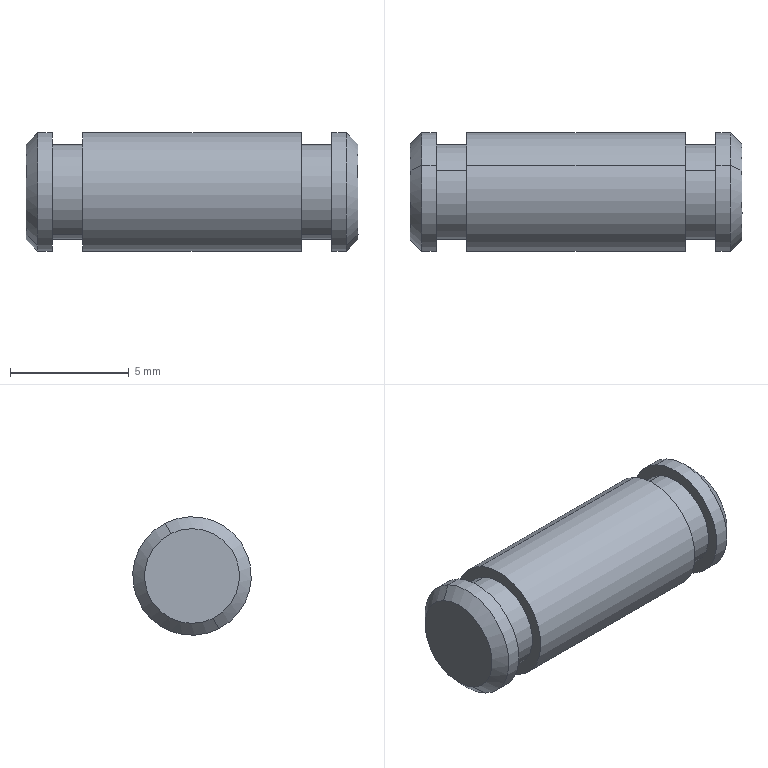Component | SolidWorks | LeverHydraulicRod22-1_HLKA-22-1 | 1 solid | 20 faces | box 14 x 5 x 5 mm | volume 253 mm3 | cylinder 10 | plane 6 | cone 4 | commonest cylinder face diameters 5 x6 4 x4
STEP:
#1=CARTESIAN_POINT('',(-2.918,4.515,-3.534));
#2=VERTEX_POINT('',#1);
#3=CARTESIAN_POINT('',(-2.918,4.426,-3.71));
#4=VERTEX_POINT('',#3);
#5=CARTESIAN_POINT('',(-2.918,4.47,-3.622));
#6=DIRECTION('',(1.,0.,0.));
#7=DIRECTION('',(0.,-0.4491,-0.8935));
#8=AXIS2_PLACEMENT_3D('',#5,#6,#7);
#9=CIRCLE('',#8,0.09843);
#10=EDGE_CURVE('',#2,#4,#9,.T.);
#11=ORIENTED_EDGE('',*,*,#10,.T.);
#12=CARTESIAN_POINT('',(-2.894,4.426,-3.71));
#13=VERTEX_POINT('',#12);
#14=CARTESIAN_POINT('',(-2.938,4.426,-3.71));
#15=DIRECTION('',(1.,0.,0.));
#16=VECTOR('',#15,39.37);
#17=LINE('',#14,#16);
#18=EDGE_CURVE('',#4,#13,#17,.T.);
#19=ORIENTED_EDGE('',*,*,#18,.T.);
#20=CARTESIAN_POINT('',(-2.894,4.515,-3.534));
#21=VERTEX_POINT('',#20);
#22=CARTESIAN_POINT('',(-2.894,4.47,-3.622));
#23=DIRECTION('',(1.,0.,0.));
#24=DIRECTION('',(0.,-0.4491,-0.8935));
#25=AXIS2_PLACEMENT_3D('',#22,#23,#24);
#26=CIRCLE('',#25,0.09843);
#27=EDGE_CURVE('',#21,#13,#26,.T.);
#28=ORIENTED_EDGE('',*,*,#27,.F.);
#29=CARTESIAN_POINT('',(-2.938,4.515,-3.534));
#30=DIRECTION('',(1.,0.,0.));
#31=VECTOR('',#30,39.37);
#32=LINE('',#29,#31);
#33=EDGE_CURVE('',#2,#21,#32,.T.);
#34=ORIENTED_EDGE('',*,*,#33,.F.);
#35=EDGE_LOOP('',(#11,#19,#28,#34));
#36=FACE_OUTER_BOUND('',#35,.T.);
#37=CARTESIAN_POINT('',(-2.938,4.47,-3.622));
#38=DIRECTION('',(1.,0.,0.));
#39=DIRECTION('',(0.,0.4491,0.8935));
#40=AXIS2_PLACEMENT_3D('',#37,#38,#39);
#41=CYLINDRICAL_SURFACE('',#40,0.09843);
#42=ADVANCED_FACE('',(#36),#41,.T.);
#43=CARTESIAN_POINT('',(-2.938,4.435,-3.692));
#44=VERTEX_POINT('',#43);
#45=CARTESIAN_POINT('',(-2.938,4.506,-3.552));
#46=VERTEX_POINT('',#45);
#47=CARTESIAN_POINT('',(-2.938,4.47,-3.622));
#48=DIRECTION('',(-1.,-0.,-0.));
#49=DIRECTION('',(0.,-0.4491,-0.8935));
#50=AXIS2_PLACEMENT_3D('',#47,#48,#49);
#51=CIRCLE('',#50,0.07874);
#52=EDGE_CURVE('',#44,#46,#51,.T.);
#53=ORIENTED_EDGE('',*,*,#52,.F.);
#54=CARTESIAN_POINT('',(-2.938,4.435,-3.692));
#55=DIRECTION('',(0.7071,-0.3176,-0.6318));
#56=VECTOR('',#55,39.37);
#57=LINE('',#54,#56);
#58=EDGE_CURVE('',#44,#4,#57,.T.);
#59=ORIENTED_EDGE('',*,*,#58,.T.);
#60=ORIENTED_EDGE('',*,*,#10,.F.);
#61=CARTESIAN_POINT('',(-2.938,4.506,-3.552));
#62=DIRECTION('',(0.7071,0.3176,0.6318));
#63=VECTOR('',#62,39.37);
#64=LINE('',#61,#63);
#65=EDGE_CURVE('',#46,#2,#64,.T.);
#66=ORIENTED_EDGE('',*,*,#65,.F.);
#67=EDGE_LOOP('',(#53,#59,#60,#66));
#68=FACE_OUTER_BOUND('',#67,.T.);
#69=CARTESIAN_POINT('',(-2.938,4.47,-3.622));
#70=DIRECTION('',(1.,0.,0.));
#71=DIRECTION('',(0.,0.4491,0.8935));
#72=AXIS2_PLACEMENT_3D('',#69,#70,#71);
#73=CONICAL_SURFACE('',#72,0.07874,0.7854);
#74=ADVANCED_FACE('',(#68),#73,.T.);
#75=CARTESIAN_POINT('',(-2.43,4.426,-3.71));
#76=VERTEX_POINT('',#75);
#77=CARTESIAN_POINT('',(-2.43,4.515,-3.534));
#78=VERTEX_POINT('',#77);
#79=CARTESIAN_POINT('',(-2.43,4.47,-3.622));
#80=DIRECTION('',(-1.,-0.,-0.));
#81=DIRECTION('',(-0.,0.4491,0.8935));
#82=AXIS2_PLACEMENT_3D('',#79,#80,#81);
#83=CIRCLE('',#82,0.09843);
#84=EDGE_CURVE('',#76,#78,#83,.T.);
#85=ORIENTED_EDGE('',*,*,#84,.F.);
#86=CARTESIAN_POINT('',(-2.406,4.426,-3.71));
#87=VERTEX_POINT('',#86);
#88=CARTESIAN_POINT('',(-2.938,4.426,-3.71));
#89=DIRECTION('',(1.,0.,0.));
#90=VECTOR('',#89,39.37);
#91=LINE('',#88,#90);
#92=EDGE_CURVE('',#76,#87,#91,.T.);
#93=ORIENTED_EDGE('',*,*,#92,.T.);
#94=CARTESIAN_POINT('',(-2.406,4.515,-3.534));
#95=VERTEX_POINT('',#94);
#96=CARTESIAN_POINT('',(-2.406,4.47,-3.622));
#97=DIRECTION('',(-1.,-0.,-0.));
#98=DIRECTION('',(0.,-0.4491,-0.8935));
#99=AXIS2_PLACEMENT_3D('',#96,#97,#98);
#100=CIRCLE('',#99,0.09843);
#101=EDGE_CURVE('',#87,#95,#100,.T.);
#102=ORIENTED_EDGE('',*,*,#101,.T.);
#103=CARTESIAN_POINT('',(-2.938,4.515,-3.534));
#104=DIRECTION('',(1.,0.,0.));
#105=VECTOR('',#104,39.37);
#106=LINE('',#103,#105);
#107=EDGE_CURVE('',#78,#95,#106,.T.);
#108=ORIENTED_EDGE('',*,*,#107,.F.);
#109=EDGE_LOOP('',(#85,#93,#102,#108));
#110=FACE_OUTER_BOUND('',#109,.T.);
#111=CARTESIAN_POINT('',(-2.938,4.47,-3.622));
#112=DIRECTION('',(1.,0.,0.));
#113=DIRECTION('',(0.,0.4491,0.8935));
#114=AXIS2_PLACEMENT_3D('',#111,#112,#113);
#115=CYLINDRICAL_SURFACE('',#114,0.09843);
#116=ADVANCED_FACE('',(#110),#115,.T.);
#117=CARTESIAN_POINT('',(-2.387,4.506,-3.552));
#118=VERTEX_POINT('',#117);
#119=CARTESIAN_POINT('',(-2.387,4.435,-3.692));
#120=VERTEX_POINT('',#119);
#121=CARTESIAN_POINT('',(-2.387,4.47,-3.622));
#122=DIRECTION('',(1.,0.,0.));
#123=DIRECTION('',(0.,-0.4491,-0.8935));
#124=AXIS2_PLACEMENT_3D('',#121,#122,#123);
#125=CIRCLE('',#124,0.07874);
#126=EDGE_CURVE('',#118,#120,#125,.T.);
#127=ORIENTED_EDGE('',*,*,#126,.F.);
#128=CARTESIAN_POINT('',(-2.406,4.515,-3.534));
#129=DIRECTION('',(-0.7071,0.3176,0.6318));
#130=VECTOR('',#129,39.37);
#131=LINE('',#128,#130);
#132=EDGE_CURVE('',#118,#95,#131,.T.);
#133=ORIENTED_EDGE('',*,*,#132,.T.);
#134=ORIENTED_EDGE('',*,*,#101,.F.);
#135=CARTESIAN_POINT('',(-2.406,4.426,-3.71));
#136=DIRECTION('',(-0.7071,-0.3176,-0.6318));
#137=VECTOR('',#136,39.37);
#138=LINE('',#135,#137);
#139=EDGE_CURVE('',#120,#87,#138,.T.);
#140=ORIENTED_EDGE('',*,*,#139,.F.);
#141=EDGE_LOOP('',(#127,#133,#134,#140));
#142=FACE_OUTER_BOUND('',#141,.T.);
#143=CARTESIAN_POINT('',(-2.406,4.47,-3.622));
#144=DIRECTION('',(-1.,-0.,-0.));
#145=DIRECTION('',(0.,-0.4491,-0.8935));
#146=AXIS2_PLACEMENT_3D('',#143,#144,#145);
#147=CONICAL_SURFACE('',#146,0.09843,0.7854);
#148=ADVANCED_FACE('',(#142),#147,.T.);
#149=CARTESIAN_POINT('',(-2.894,4.506,-3.552));
#150=VERTEX_POINT('',#149);
#151=CARTESIAN_POINT('',(-2.894,4.435,-3.692));
#152=VERTEX_POINT('',#151);
#153=CARTESIAN_POINT('',(-2.894,4.47,-3.622));
#154=DIRECTION('',(1.,0.,0.));
#155=DIRECTION('',(0.,0.4491,0.8935));
#156=AXIS2_PLACEMENT_3D('',#153,#154,#155);
#157=CIRCLE('',#156,0.07874);
#158=EDGE_CURVE('',#150,#152,#157,.T.);
#159=ORIENTED_EDGE('',*,*,#158,.T.);
#160=CARTESIAN_POINT('',(-2.843,4.435,-3.692));
#161=VERTEX_POINT('',#160);
#162=CARTESIAN_POINT('',(-2.387,4.435,-3.692));
#163=DIRECTION('',(1.,0.,0.));
#164=VECTOR('',#163,39.37);
#165=LINE('',#162,#164);
#166=EDGE_CURVE('',#152,#161,#165,.T.);
#167=ORIENTED_EDGE('',*,*,#166,.T.);
#168=CARTESIAN_POINT('',(-2.843,4.506,-3.552));
#169=VERTEX_POINT('',#168);
#170=CARTESIAN_POINT('',(-2.843,4.47,-3.622));
#171=DIRECTION('',(1.,0.,0.));
#172=DIRECTION('',(0.,0.4491,0.8935));
#173=AXIS2_PLACEMENT_3D('',#170,#171,#172);
#174=CIRCLE('',#173,0.07874);
#175=EDGE_CURVE('',#169,#161,#174,.T.);
#176=ORIENTED_EDGE('',*,*,#175,.F.);
#177=CARTESIAN_POINT('',(-2.387,4.506,-3.552));
#178=DIRECTION('',(1.,0.,0.));
#179=VECTOR('',#178,39.37);
#180=LINE('',#177,#179);
#181=EDGE_CURVE('',#150,#169,#180,.T.);
#182=ORIENTED_EDGE('',*,*,#181,.F.);
#183=EDGE_LOOP('',(#159,#167,#176,#182));
#184=FACE_OUTER_BOUND('',#183,.T.);
#185=CARTESIAN_POINT('',(-2.387,4.47,-3.622));
#186=DIRECTION('',(1.,0.,0.));
#187=DIRECTION('',(-0.,0.4491,0.8935));
#188=AXIS2_PLACEMENT_3D('',#185,#186,#187);
#189=CYLINDRICAL_SURFACE('',#188,0.07874);
#190=ADVANCED_FACE('',(#184),#189,.T.);
#191=CARTESIAN_POINT('',(-2.481,4.506,-3.552));
#192=VERTEX_POINT('',#191);
#193=CARTESIAN_POINT('',(-2.481,4.435,-3.692));
#194=VERTEX_POINT('',#193);
#195=CARTESIAN_POINT('',(-2.481,4.47,-3.622));
#196=DIRECTION('',(1.,0.,0.));
#197=DIRECTION('',(0.,0.4491,0.8935));
#198=AXIS2_PLACEMENT_3D('',#195,#196,#197);
#199=CIRCLE('',#198,0.07874);
#200=EDGE_CURVE('',#192,#194,#199,.T.);
#201=ORIENTED_EDGE('',*,*,#200,.T.);
#202=CARTESIAN_POINT('',(-2.43,4.435,-3.692));
#203=VERTEX_POINT('',#202);
#204=CARTESIAN_POINT('',(-2.387,4.435,-3.692));
#205=DIRECTION('',(1.,0.,0.));
#206=VECTOR('',#205,39.37);
#207=LINE('',#204,#206);
#208=EDGE_CURVE('',#194,#203,#207,.T.);
#209=ORIENTED_EDGE('',*,*,#208,.T.);
#210=CARTESIAN_POINT('',(-2.43,4.506,-3.552));
#211=VERTEX_POINT('',#210);
#212=CARTESIAN_POINT('',(-2.43,4.47,-3.622));
#213=DIRECTION('',(1.,0.,0.));
#214=DIRECTION('',(-0.,0.4491,0.8935));
#215=AXIS2_PLACEMENT_3D('',#212,#213,#214);
#216=CIRCLE('',#215,0.07874);
#217=EDGE_CURVE('',#211,#203,#216,.T.);
#218=ORIENTED_EDGE('',*,*,#217,.F.);
#219=CARTESIAN_POINT('',(-2.387,4.506,-3.552));
#220=DIRECTION('',(1.,0.,0.));
#221=VECTOR('',#220,39.37);
#222=LINE('',#219,#221);
#223=EDGE_CURVE('',#192,#211,#222,.T.);
#224=ORIENTED_EDGE('',*,*,#223,.F.);
#225=EDGE_LOOP('',(#201,#209,#218,#224));
#226=FACE_OUTER_BOUND('',#225,.T.);
#227=CARTESIAN_POINT('',(-2.387,4.47,-3.622));
#228=DIRECTION('',(1.,0.,0.));
#229=DIRECTION('',(-0.,0.4491,0.8935));
#230=AXIS2_PLACEMENT_3D('',#227,#228,#229);
#231=CYLINDRICAL_SURFACE('',#230,0.07874);
#232=ADVANCED_FACE('',(#226),#231,.T.);
#233=CARTESIAN_POINT('',(-2.843,4.515,-3.534));
#234=VERTEX_POINT('',#233);
#235=CARTESIAN_POINT('',(-2.843,4.426,-3.71));
#236=VERTEX_POINT('',#235);
#237=CARTESIAN_POINT('',(-2.843,4.47,-3.622));
#238=DIRECTION('',(1.,0.,0.));
#239=DIRECTION('',(0.,0.4491,0.8935));
#240=AXIS2_PLACEMENT_3D('',#237,#238,#239);
#241=CIRCLE('',#240,0.09843);
#242=EDGE_CURVE('',#234,#236,#241,.T.);
#243=ORIENTED_EDGE('',*,*,#242,.T.);
#244=CARTESIAN_POINT('',(-2.481,4.426,-3.71));
#245=VERTEX_POINT('',#244);
#246=CARTESIAN_POINT('',(-2.938,4.426,-3.71));
#247=DIRECTION('',(1.,0.,0.));
#248=VECTOR('',#247,39.37);
#249=LINE('',#246,#248);
#250=EDGE_CURVE('',#236,#245,#249,.T.);
#251=ORIENTED_EDGE('',*,*,#250,.T.);
#252=CARTESIAN_POINT('',(-2.481,4.515,-3.534));
#253=VERTEX_POINT('',#252);
#254=CARTESIAN_POINT('',(-2.481,4.47,-3.622));
#255=DIRECTION('',(-1.,-0.,-0.));
#256=DIRECTION('',(0.,-0.4491,-0.8935));
#257=AXIS2_PLACEMENT_3D('',#254,#255,#256);
#258=CIRCLE('',#257,0.09843);
#259=EDGE_CURVE('',#245,#253,#258,.T.);
#260=ORIENTED_EDGE('',*,*,#259,.T.);
#261=CARTESIAN_POINT('',(-2.938,4.515,-3.534));
#262=DIRECTION('',(1.,0.,0.));
#263=VECTOR('',#262,39.37);
#264=LINE('',#261,#263);
#265=EDGE_CURVE('',#234,#253,#264,.T.);
#266=ORIENTED_EDGE('',*,*,#265,.F.);
#267=EDGE_LOOP('',(#243,#251,#260,#266));
#268=FACE_OUTER_BOUND('',#267,.T.);
#269=CARTESIAN_POINT('',(-2.938,4.47,-3.622));
#270=DIRECTION('',(1.,0.,0.));
#271=DIRECTION('',(0.,0.4491,0.8935));
#272=AXIS2_PLACEMENT_3D('',#269,#270,#271);
#273=CYLINDRICAL_SURFACE('',#272,0.09843);
#274=ADVANCED_FACE('',(#268),#273,.T.);
#275=ORIENTED_EDGE('',*,*,#175,.T.);
#276=CARTESIAN_POINT('',(-2.843,4.47,-3.622));
#277=DIRECTION('',(1.,0.,0.));
#278=DIRECTION('',(0.,0.4491,0.8935));
#279=AXIS2_PLACEMENT_3D('',#276,#277,#278);
#280=CIRCLE('',#279,0.07874);
#281=EDGE_CURVE('',#161,#169,#280,.T.);
#282=ORIENTED_EDGE('',*,*,#281,.T.);
#283=EDGE_LOOP('',(#275,#282));
#284=FACE_BOUND('',#283,.T.);
#285=ORIENTED_EDGE('',*,*,#242,.F.);
#286=CARTESIAN_POINT('',(-2.843,4.47,-3.622));
#287=DIRECTION('',(1.,0.,0.));
#288=DIRECTION('',(0.,0.4491,0.8935));
#289=AXIS2_PLACEMENT_3D('',#286,#287,#288);
#290=CIRCLE('',#289,0.09843);
#291=EDGE_CURVE('',#236,#234,#290,.T.);
#292=ORIENTED_EDGE('',*,*,#291,.F.);
#293=EDGE_LOOP('',(#285,#292));
#294=FACE_OUTER_BOUND('',#293,.T.);
#295=CARTESIAN_POINT('',(-2.843,4.543,-3.478));
#296=DIRECTION('',(1.,-0.,0.));
#297=DIRECTION('',(0.,0.8935,-0.4491));
#298=AXIS2_PLACEMENT_3D('',#295,#296,#297);
#299=PLANE('',#298);
#300=ADVANCED_FACE('',(#284,#294),#299,.F.);
#301=ORIENTED_EDGE('',*,*,#200,.F.);
#302=CARTESIAN_POINT('',(-2.481,4.47,-3.622));
#303=DIRECTION('',(1.,0.,0.));
#304=DIRECTION('',(0.,0.4491,0.8935));
#305=AXIS2_PLACEMENT_3D('',#302,#303,#304);
#306=CIRCLE('',#305,0.07874);
#307=EDGE_CURVE('',#194,#192,#306,.T.);
#308=ORIENTED_EDGE('',*,*,#307,.F.);
#309=EDGE_LOOP('',(#301,#308));
#310=FACE_BOUND('',#309,.T.);
#311=CARTESIAN_POINT('',(-2.481,4.47,-3.622));
#312=DIRECTION('',(-1.,-0.,-0.));
#313=DIRECTION('',(0.,-0.4491,-0.8935));
#314=AXIS2_PLACEMENT_3D('',#311,#312,#313);
#315=CIRCLE('',#314,0.09843);
#316=EDGE_CURVE('',#253,#245,#315,.T.);
#317=ORIENTED_EDGE('',*,*,#316,.F.);
#318=ORIENTED_EDGE('',*,*,#259,.F.);
#319=EDGE_LOOP('',(#317,#318));
#320=FACE_OUTER_BOUND('',#319,.T.);
#321=CARTESIAN_POINT('',(-2.481,4.538,-3.487));
#322=DIRECTION('',(-1.,-0.,-0.));
#323=DIRECTION('',(0.,-0.4491,-0.8935));
#324=AXIS2_PLACEMENT_3D('',#321,#322,#323);
#325=PLANE('',#324);
#326=ADVANCED_FACE('',(#310,#320),#325,.F.);
#327=ORIENTED_EDGE('',*,*,#250,.F.);
#328=ORIENTED_EDGE('',*,*,#291,.T.);
#329=ORIENTED_EDGE('',*,*,#265,.T.);
#330=ORIENTED_EDGE('',*,*,#316,.T.);
#331=EDGE_LOOP('',(#327,#328,#329,#330));
#332=FACE_OUTER_BOUND('',#331,.T.);
#333=CARTESIAN_POINT('',(-2.938,4.47,-3.622));
#334=DIRECTION('',(1.,0.,0.));
#335=DIRECTION('',(0.,0.4491,0.8935));
#336=AXIS2_PLACEMENT_3D('',#333,#334,#335);
#337=CYLINDRICAL_SURFACE('',#336,0.09843);
#338=ADVANCED_FACE('',(#332),#337,.T.);
#339=ORIENTED_EDGE('',*,*,#208,.F.);
#340=ORIENTED_EDGE('',*,*,#307,.T.);
#341=ORIENTED_EDGE('',*,*,#223,.T.);
#342=CARTESIAN_POINT('',(-2.43,4.47,-3.622));
#343=DIRECTION('',(1.,0.,0.));
#344=DIRECTION('',(-0.,0.4491,0.8935));
#345=AXIS2_PLACEMENT_3D('',#342,#343,#344);
#346=CIRCLE('',#345,0.07874);
#347=EDGE_CURVE('',#203,#211,#346,.T.);
#348=ORIENTED_EDGE('',*,*,#347,.F.);
#349=EDGE_LOOP('',(#339,#340,#341,#348));
#350=FACE_OUTER_BOUND('',#349,.T.);
#351=CARTESIAN_POINT('',(-2.387,4.47,-3.622));
#352=DIRECTION('',(1.,0.,0.));
#353=DIRECTION('',(-0.,0.4491,0.8935));
#354=AXIS2_PLACEMENT_3D('',#351,#352,#353);
#355=CYLINDRICAL_SURFACE('',#354,0.07874);
#356=ADVANCED_FACE('',(#350),#355,.T.);
#357=ORIENTED_EDGE('',*,*,#166,.F.);
#358=CARTESIAN_POINT('',(-2.894,4.47,-3.622));
#359=DIRECTION('',(1.,0.,0.));
#360=DIRECTION('',(0.,0.4491,0.8935));
#361=AXIS2_PLACEMENT_3D('',#358,#359,#360);
#362=CIRCLE('',#361,0.07874);
#363=EDGE_CURVE('',#152,#150,#362,.T.);
#364=ORIENTED_EDGE('',*,*,#363,.T.);
#365=ORIENTED_EDGE('',*,*,#181,.T.);
#366=ORIENTED_EDGE('',*,*,#281,.F.);
#367=EDGE_LOOP('',(#357,#364,#365,#366));
#368=FACE_OUTER_BOUND('',#367,.T.);
#369=CARTESIAN_POINT('',(-2.387,4.47,-3.622));
#370=DIRECTION('',(1.,0.,0.));
#371=DIRECTION('',(-0.,0.4491,0.8935));
#372=AXIS2_PLACEMENT_3D('',#369,#370,#371);
#373=CYLINDRICAL_SURFACE('',#372,0.07874);
#374=ADVANCED_FACE('',(#368),#373,.T.);
#375=CARTESIAN_POINT('',(-2.43,4.47,-3.622));
#376=DIRECTION('',(-1.,-0.,-0.));
#377=DIRECTION('',(-0.,0.4491,0.8935));
#378=AXIS2_PLACEMENT_3D('',#375,#376,#377);
#379=CIRCLE('',#378,0.09843);
#380=EDGE_CURVE('',#78,#76,#379,.T.);
#381=ORIENTED_EDGE('',*,*,#380,.T.);
#382=ORIENTED_EDGE('',*,*,#84,.T.);
#383=EDGE_LOOP('',(#381,#382));
#384=FACE_OUTER_BOUND('',#383,.T.);
#385=ORIENTED_EDGE('',*,*,#217,.T.);
#386=ORIENTED_EDGE('',*,*,#347,.T.);
#387=EDGE_LOOP('',(#385,#386));
#388=FACE_BOUND('',#387,.T.);
#389=CARTESIAN_POINT('',(-2.43,4.365,-3.569));
#390=DIRECTION('',(1.,0.,0.));
#391=DIRECTION('',(-0.,0.4491,0.8935));
#392=AXIS2_PLACEMENT_3D('',#389,#390,#391);
#393=PLANE('',#392);
#394=ADVANCED_FACE('',(#384,#388),#393,.F.);
#395=CARTESIAN_POINT('',(-2.387,4.47,-3.622));
#396=DIRECTION('',(1.,0.,0.));
#397=DIRECTION('',(0.,-0.4491,-0.8935));
#398=AXIS2_PLACEMENT_3D('',#395,#396,#397);
#399=CIRCLE('',#398,0.07874);
#400=EDGE_CURVE('',#120,#118,#399,.T.);
#401=ORIENTED_EDGE('',*,*,#400,.T.);
#402=ORIENTED_EDGE('',*,*,#126,.T.);
#403=EDGE_LOOP('',(#401,#402));
#404=FACE_OUTER_BOUND('',#403,.T.);
#405=CARTESIAN_POINT('',(-2.387,4.47,-3.622));
#406=DIRECTION('',(-1.,-0.,-0.));
#407=DIRECTION('',(0.,-0.4491,-0.8935));
#408=AXIS2_PLACEMENT_3D('',#405,#406,#407);
#409=PLANE('',#408);
#410=ADVANCED_FACE('',(#404),#409,.F.);
#411=ORIENTED_EDGE('',*,*,#132,.F.);
#412=ORIENTED_EDGE('',*,*,#400,.F.);
#413=ORIENTED_EDGE('',*,*,#139,.T.);
#414=CARTESIAN_POINT('',(-2.406,4.47,-3.622));
#415=DIRECTION('',(-1.,-0.,-0.));
#416=DIRECTION('',(0.,-0.4491,-0.8935));
#417=AXIS2_PLACEMENT_3D('',#414,#415,#416);
#418=CIRCLE('',#417,0.09843);
#419=EDGE_CURVE('',#95,#87,#418,.T.);
#420=ORIENTED_EDGE('',*,*,#419,.F.);
#421=EDGE_LOOP('',(#411,#412,#413,#420));
#422=FACE_OUTER_BOUND('',#421,.T.);
#423=CARTESIAN_POINT('',(-2.406,4.47,-3.622));
#424=DIRECTION('',(-1.,-0.,-0.));
#425=DIRECTION('',(0.,-0.4491,-0.8935));
#426=AXIS2_PLACEMENT_3D('',#423,#424,#425);
#427=CONICAL_SURFACE('',#426,0.09843,0.7854);
#428=ADVANCED_FACE('',(#422),#427,.T.);
#429=ORIENTED_EDGE('',*,*,#92,.F.);
#430=ORIENTED_EDGE('',*,*,#380,.F.);
#431=ORIENTED_EDGE('',*,*,#107,.T.);
#432=ORIENTED_EDGE('',*,*,#419,.T.);
#433=EDGE_LOOP('',(#429,#430,#431,#432));
#434=FACE_OUTER_BOUND('',#433,.T.);
#435=CARTESIAN_POINT('',(-2.938,4.47,-3.622));
#436=DIRECTION('',(1.,0.,0.));
#437=DIRECTION('',(0.,0.4491,0.8935));
#438=AXIS2_PLACEMENT_3D('',#435,#436,#437);
#439=CYLINDRICAL_SURFACE('',#438,0.09843);
#440=ADVANCED_FACE('',(#434),#439,.T.);
#441=ORIENTED_EDGE('',*,*,#27,.T.);
#442=CARTESIAN_POINT('',(-2.894,4.47,-3.622));
#443=DIRECTION('',(1.,0.,0.));
#444=DIRECTION('',(0.,-0.4491,-0.8935));
#445=AXIS2_PLACEMENT_3D('',#442,#443,#444);
#446=CIRCLE('',#445,0.09843);
#447=EDGE_CURVE('',#13,#21,#446,.T.);
#448=ORIENTED_EDGE('',*,*,#447,.T.);
#449=EDGE_LOOP('',(#441,#448));
#450=FACE_OUTER_BOUND('',#449,.T.);
#451=ORIENTED_EDGE('',*,*,#158,.F.);
#452=ORIENTED_EDGE('',*,*,#363,.F.);
#453=EDGE_LOOP('',(#451,#452));
#454=FACE_BOUND('',#453,.T.);
#455=CARTESIAN_POINT('',(-2.894,4.4,-3.587));
#456=DIRECTION('',(-1.,-0.,-0.));
#457=DIRECTION('',(0.,-0.4491,-0.8935));
#458=AXIS2_PLACEMENT_3D('',#455,#456,#457);
#459=PLANE('',#458);
#460=ADVANCED_FACE('',(#450,#454),#459,.F.);
#461=CARTESIAN_POINT('',(-2.938,4.47,-3.622));
#462=DIRECTION('',(-1.,-0.,-0.));
#463=DIRECTION('',(0.,-0.4491,-0.8935));
#464=AXIS2_PLACEMENT_3D('',#461,#462,#463);
#465=CIRCLE('',#464,0.07874);
#466=EDGE_CURVE('',#46,#44,#465,.T.);
#467=ORIENTED_EDGE('',*,*,#466,.T.);
#468=ORIENTED_EDGE('',*,*,#52,.T.);
#469=EDGE_LOOP('',(#467,#468));
#470=FACE_OUTER_BOUND('',#469,.T.);
#471=CARTESIAN_POINT('',(-2.938,4.47,-3.622));
#472=DIRECTION('',(-1.,-0.,-0.));
#473=DIRECTION('',(0.,-0.4491,-0.8935));
#474=AXIS2_PLACEMENT_3D('',#471,#472,#473);
#475=PLANE('',#474);
#476=ADVANCED_FACE('',(#470),#475,.T.);
#477=ORIENTED_EDGE('',*,*,#58,.F.);
#478=ORIENTED_EDGE('',*,*,#466,.F.);
#479=ORIENTED_EDGE('',*,*,#65,.T.);
#480=CARTESIAN_POINT('',(-2.918,4.47,-3.622));
#481=DIRECTION('',(1.,0.,0.));
#482=DIRECTION('',(0.,-0.4491,-0.8935));
#483=AXIS2_PLACEMENT_3D('',#480,#481,#482);
#484=CIRCLE('',#483,0.09843);
#485=EDGE_CURVE('',#4,#2,#484,.T.);
#486=ORIENTED_EDGE('',*,*,#485,.F.);
#487=EDGE_LOOP('',(#477,#478,#479,#486));
#488=FACE_OUTER_BOUND('',#487,.T.);
#489=CARTESIAN_POINT('',(-2.938,4.47,-3.622));
#490=DIRECTION('',(1.,0.,0.));
#491=DIRECTION('',(0.,0.4491,0.8935));
#492=AXIS2_PLACEMENT_3D('',#489,#490,#491);
#493=CONICAL_SURFACE('',#492,0.07874,0.7854);
#494=ADVANCED_FACE('',(#488),#493,.T.);
#495=ORIENTED_EDGE('',*,*,#18,.F.);
#496=ORIENTED_EDGE('',*,*,#485,.T.);
#497=ORIENTED_EDGE('',*,*,#33,.T.);
#498=ORIENTED_EDGE('',*,*,#447,.F.);
#499=EDGE_LOOP('',(#495,#496,#497,#498));
#500=FACE_OUTER_BOUND('',#499,.T.);
#501=CARTESIAN_POINT('',(-2.938,4.47,-3.622));
#502=DIRECTION('',(1.,0.,0.));
#503=DIRECTION('',(0.,0.4491,0.8935));
#504=AXIS2_PLACEMENT_3D('',#501,#502,#503);
#505=CYLINDRICAL_SURFACE('',#504,0.09843);
#506=ADVANCED_FACE('',(#500),#505,.T.);
#507=CLOSED_SHELL('',(#42,#74,#116,#148,#190,#232,#274,#300,#326,#338,#356,#374,#394,#410,#428,#440,#460,#476,#494,#506));
#508=MANIFOLD_SOLID_BREP('',#507);
#509=CARTESIAN_POINT('',(0.,0.,0.));
#510=DIRECTION('',(0.,0.,1.));
#511=DIRECTION('',(1.,0.,0.));
#512=AXIS2_PLACEMENT_3D('',#509,#510,#511);
#513=(LENGTH_UNIT()NAMED_UNIT(*)SI_UNIT($,.METRE.));
#514=LENGTH_MEASURE_WITH_UNIT(LENGTH_MEASURE(0.0254),#513);
#515=DIMENSIONAL_EXPONENTS(1.,0.,0.,0.,0.,0.,0.);
#516=(CONVERSION_BASED_UNIT('',#514)LENGTH_UNIT()NAMED_UNIT(#515));
#517=UNCERTAINTY_MEASURE_WITH_UNIT(LENGTH_MEASURE(0.00001),#516,'','');
#518=(NAMED_UNIT(*)PLANE_ANGLE_UNIT()SI_UNIT($,.RADIAN.));
#519=(NAMED_UNIT(*)SI_UNIT($,.STERADIAN.)SOLID_ANGLE_UNIT());
#520=(GEOMETRIC_REPRESENTATION_CONTEXT(3)GLOBAL_UNCERTAINTY_ASSIGNED_CONTEXT((#517))GLOBAL_UNIT_ASSIGNED_CONTEXT((#516,#518,#519))REPRESENTATION_CONTEXT('',''));
#521=ADVANCED_BREP_SHAPE_REPRESENTATION('',(#508,#512),#520);
#522=COLOUR_RGB('',0.7922,0.8196,0.9333);
#523=FILL_AREA_STYLE_COLOUR('',#522);
#524=FILL_AREA_STYLE('',(#523));
#525=SURFACE_STYLE_FILL_AREA(#524);
#526=SURFACE_SIDE_STYLE('',(#525));
#527=SURFACE_STYLE_USAGE(.BOTH.,#526);
#528=PRESENTATION_STYLE_ASSIGNMENT((#527));
#529=STYLED_ITEM('',(#528),#508);
#530=(LENGTH_UNIT()NAMED_UNIT(*)SI_UNIT($,.METRE.));
#531=LENGTH_MEASURE_WITH_UNIT(LENGTH_MEASURE(0.0254),#530);
#532=DIMENSIONAL_EXPONENTS(1.,0.,0.,0.,0.,0.,0.);
#533=(CONVERSION_BASED_UNIT('',#531)LENGTH_UNIT()NAMED_UNIT(#532));
#534=UNCERTAINTY_MEASURE_WITH_UNIT(LENGTH_MEASURE(0.00001),#533,'','');
#535=(NAMED_UNIT(*)PLANE_ANGLE_UNIT()SI_UNIT($,.RADIAN.));
#536=(NAMED_UNIT(*)SI_UNIT($,.STERADIAN.)SOLID_ANGLE_UNIT());
#537=(GEOMETRIC_REPRESENTATION_CONTEXT(3)GLOBAL_UNCERTAINTY_ASSIGNED_CONTEXT((#534))GLOBAL_UNIT_ASSIGNED_CONTEXT((#533,#535,#536))REPRESENTATION_CONTEXT('',''));
#538=MECHANICAL_DESIGN_GEOMETRIC_PRESENTATION_REPRESENTATION('',(#529),#537);
#539=PRESENTATION_LAYER_ASSIGNMENT('','',(#529));